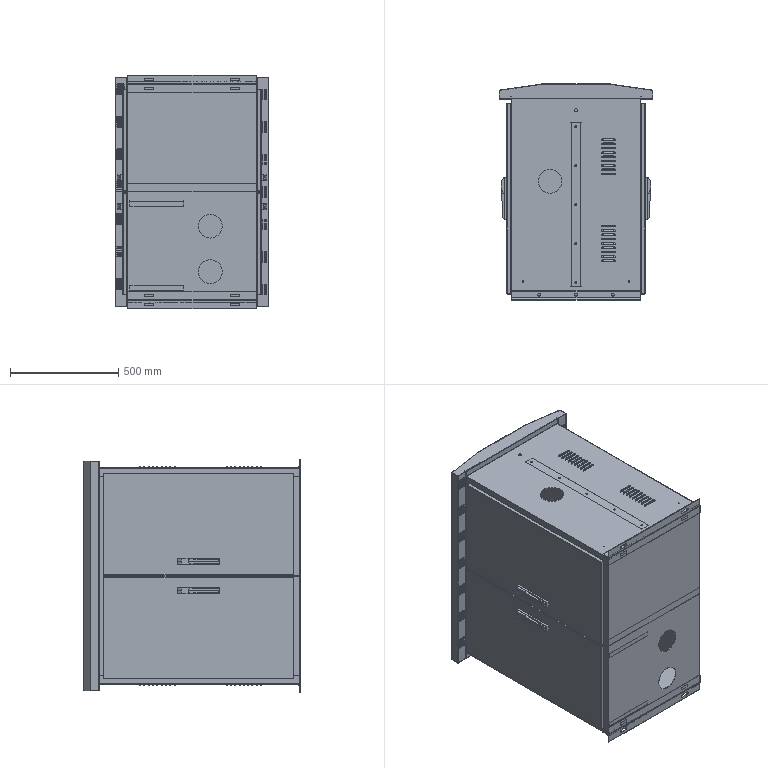Assembly | SolidWorks | mm | 61 component files | 65 solids | 4519 faces | box 710 x 1000 x 1080 mm | volume 12516403 mm3 | plane 2101 | cylinder 1978 | torus 176 | sphere 144 | spline 72 | cone 48 | commonest cylinder face diameters 4.5 x344 5.5 x332 4 x288 6 x222 4.473 x98 1.473 x98 9 x86 12 x56
Bill of materials:
CompensationChamberDoorPanel | 1 |  | Thin rectangular sheet panel with short perimeter return flanges; one large rectangular cutout near the top and a pattern of round holes below it.
CompositeSwitchMountingBeam100 | 2 |  | Long, narrow formed sheet bracket with a U/channel-type cross-section and flat extended end tabs, each tab carrying two elongated slots.
FrameLongitudinalBeamFive100 | 1 |  | Long open U-channel (open side up) formed from sheet, with pairs of small holes along both side walls.
FrameLongitudinalBeamFour01100 | 1 |  | Long open U-channel formed from sheet, with paired small holes along the side walls and holes near each end of the web.
FrameLongitudinalBeamOne01100 | 1 |  | Long L-section angle formed from sheet; one leg has five evenly spaced elongated slots, and that leg is slightly shorter than the other with trimmed corners at its ends.
FrameLongitudinalBeamSix100 | 1 |  | Long inverted U-channel (open side down) formed from sheet, with two holes at each end of the web and paired small holes along the side walls.
FrameLongitudinalBeamThree40001100 | 1 |  | Long plain L-section angle with a rounded bend; one leg carries five evenly spaced elongated slots.
FrameLongitudinalBeamTwo40001100 | 1 |  | Long inverted U-channel formed from sheet, with a row of evenly spaced round holes along the web and paired small holes along the side walls.
FrameTransverseBeamOne40001100 | 2 |  | Short, deep U-channel formed from sheet with rounded bends and rounded wall corners; two round holes near each end of one side wall.
FrameTransverseBeamTwo40001100 | 2 |  | Long, narrow formed sheet bracket with a hat/inverted-U profile and flat extended end tabs, each tab having two elongated slots; multiple round holes along the web.
FrontLeftDoorPanel100 | 1 |  | Thin flat rectangular plate with one rectangular slot near the centre of one long edge, flanked by two small round holes.
MS830-Lock | 4 | Plain Carbon Steel | Elongated solid, lever- or block-like body with a longitudinal groove along its length, a cylindrical boss partway along, a tapered section, and an angled/chamfered end.
FrontRightDoorPanel100 | 1 |  | Flat rectangular plate with a single rectangular slot near one long edge, centered along it, with one small round hole on each side of the slot.
FrontSealingPlate100 | 1 |  | Long, narrow, thin sheet panel. Both short ends have a slight downward bend or short lip. It has four larger round holes in a row near one end and four small corner holes, two at each end.
FuseGroupMountingBeam100 | 1 |  | Long U-channel bracket with rounded bend corners. The web extends past the flanges at both ends as flat tabs, and each tab has two elongated slots. Pairs of small round holes are spaced along the web.
GroundWireFixingBeam100 | 1 |  | Long U-channel bracket with rounded bends and extended end tabs, each tab with two elongated slots. Three larger round holes run along the web centerline, and one flange has a row of five small holes.
GB_INTERCHANGEABLE_PARTS_TM_EAI 4X4X594 | 4 |  | Straight, long angle-section (L-profile) bar with two legs that look equal. One leg has three round through-holes spaced along its length. The other leg has two slots, elongated along the length, one near each end.
InsulatorSYZ9-10Q100 | 4 |  | Solid body of revolution, roughly barrel-shaped. A raised cylindrical band in the middle sits between two tapered (frustum) ends, and each end face has a small central hole. The edges are slightly rounded.
LeftSidePlate400AType40001100 | 1 |  | Shallow rectangular sheet tray. Upturned side walls run along two opposite edges and end in small outward lips. The base has two groups of parallel louvers and one small round hole.
LowerCrossbar400AType40001100 | 1 |  | Sheet panel with a hat-shaped section: a flat web, two side walls bent at right angles, and short outward flanges. Both side walls have a rectangular notch at the same position partway along their length. Two large round holes sit near one side of the web.
MeteringChamberDoorPanel | 1 |  | Rectangular plate with four rectangular cutouts: one in the upper left and three stacked in a column on the right. It also has a small round hole near the top center and a pattern of one central hole with four small holes arranged in a cross around it.
MeteringChamberPartition400AType40001100 | 1 |  | Very thin flat rectangular plate with rounded corners. Three large round holes run in a column near one short edge. Small elongated slots run along both long edges, and four small round holes form a rectangular pattern.
MiddleCrossbar400AType40001100 | 2 |  | Long straight profile with a constant lipped C-channel section: a flat web, two flanges, and inward-angled lips with rounded ends. No holes are visible.
MoldedCaseMountingBeamOne100 | 4 |  | Long U-channel bracket with extended end tabs, each tab with two elongated slots. One flange has five small holes and the web has two small holes. A cylindrical boss with a chamfered end projects from the web into the inside of the channel.
MoldedCaseMountingBeamThree100 | 2 |  | Long U-channel bracket with rounded bends and extended end tabs, each tab with two elongated slots. The web has three pairs of small round holes along its centerline.
MoldedCaseMountingBeamTwo100 | 2 |  | Long, narrow formed channel (C-section) with rounded bends. The web is extended at both ends into tabs, and each tab has two slotted holes. Small round holes run along the web and the flange.
OutputN01400AType40001100 | 2 |  | Hat-profile formed bracket. Two outer mounting flanges are joined by short legs to an offset central web. Each flange has one round hole and the web has three.
RearCoverPlate100 | 1 |  | Thin, long rectangular plate with very shallow edge lips along the long sides. It has four small holes near the corners and a row of four larger round holes near one end.
RearLeftDoorPanel100 | 1 |  | Rectangular panel with a shallow folded perimeter edge (tray-like). It has a rectangular slot near one long edge, with a small round hole on each side of the slot.
RearRightDoorPanel100 | 1 |  | Rectangular panel with a shallow folded perimeter edge. It has a rectangular slot near the opposite long edge from unnamed part, with a small hole on each side.
RightSidePlate400AType40001100 | 1 |  | Shallow rectangular box-shaped cover with folded side walls. The top face has one large circular hole, one small hole, and two groups of parallel louvers or slots. Short flanges stick out past the walls along the long sides.
SmallDoorFrameOne100 | 4 |  | Long formed strip with a constant cross-section. The profile steps through several rounded bends: a hemmed J-hook at one end, two offset steps, and an upturned flange at the other end.
SmallDoorFrameTwo100 | 2 |  | Formed strip with the same kind of stepped multi-bend profile as unnamed part (hooked hem, two offsets, end flange), shown as a shorter piece.
TopCover01100 | 1 |  | Large formed panel with a faceted, arched cross-section (a central flat and two angled facets). Both side edges turn into narrow return flanges with small lips, and these returns carry repeated groups of small parallel slots or louvers.
TopCoverPlug01100 | 2 |  | Long formed strip with a flat top whose outline tapers at both ends (faceted, elongated hexagonal outline). A downturned leg runs along one edge and ends in a short stepped return.
UpperCrossbarFront400AType40001100 | 1 |  | Long L-angle with a rounded bend. One flange has a small rectangular notch at about mid-length.
UpperCrossbarRear400AType40001100 | 1 |  | Long L-angle with a rounded bend, oriented opposite to unnamed part. One flange has a small rectangular notch at about mid-length.
Mates:
1. coincident | LeftSidePlate400AType40001100-3 face at (890.554, 1085, -1.5) dir (0, 1, 0) | RightSidePlate400AType40001100-2 face at (293.554, 1085, 998.5) dir (0, 1, 0)
2. coincident | LeftSidePlate400AType40001100-3 face at (892.054, 1085, 0) dir (1, 0, 0) | RightSidePlate400AType40001100-2 face at (892.054, 1085, 958.5) dir (1, 0, 0)
3. coincident | LeftSidePlate400AType40001100-3 face at (292.054, 1085, 38.5) dir (-1, 0, 0) | UpperCrossbarRear400AType40001100-1 face at (292.054, 1087, 958.5) dir (-1, 0, 0)
4. width | LeftSidePlate400AType40001100-3 face at (890.554, 147, -1.5) dir (0, 0, -1) | RightSidePlate400AType40001100-2 face at (293.554, 147, 998.5) dir (0, 0, 1) | UpperCrossbarRear400AType40001100-1 face at (293.554, 1037, 958.5) dir (0, 0, 1) | UpperCrossbarRear400AType40001100-1 face at (293.554, 1037, 38.5) dir (0, 0, -1)
5. coincident | LeftSidePlate400AType40001100-3 face at (892.054, 1085, 0) dir (1, 0, 0) | UpperCrossbarFront400AType40001100-2 face at (892.054, 1087, 38.5) dir (1, 0, 0)
6. width | RightSidePlate400AType40001100-2 face at (293.554, 147, 998.5) dir (0, 0, 1) | LeftSidePlate400AType40001100-3 face at (890.554, 147, -1.5) dir (0, 0, -1) | UpperCrossbarFront400AType40001100-2 face at (890.554, 1037, 958.5) dir (0, 0, 1) | UpperCrossbarFront400AType40001100-2 face at (890.554, 1037, 38.5) dir (0, 0, -1)
7. coincident | LowerCrossbar400AType40001100-1 face at (292.054, 147, 38.5) dir (0, -1, 0) | RightSidePlate400AType40001100-2 face at (889.818, 147, 958.5) dir (0, -1, 0)
8. width | LeftSidePlate400AType40001100-3 face at (890.554, 147, -1.5) dir (0, 0, -1) | RightSidePlate400AType40001100-2 face at (293.554, 147, 998.5) dir (0, 0, 1) | LowerCrossbar400AType40001100-1 face at (892.054, 148.5, 958.5) dir (0, 0, 1) | LowerCrossbar400AType40001100-1 face at (892.054, 148.5, 38.5) dir (0, 0, -1)
9. width | RightSidePlate400AType40001100-2 face at (892.054, 1085, 958.5) dir (1, 0, 0) | RightSidePlate400AType40001100-2 face at (292.054, 1085, 997) dir (-1, 0, 0) | LowerCrossbar400AType40001100-1 face at (892.054, 148.5, 38.5) dir (1, 0, 0) | LowerCrossbar400AType40001100-1 face at (292.054, 148.5, 958.5) dir (-1, 0, 0)
10. width | TopCover01100-2/TopCoverPlug01100-1 face at (292.054, 1078.5, 1028.5) dir (0, 0, 1) | TopCover01100-2/TopCoverPlug01100-2 face at (892.054, 1078.5, -31.5) dir (0, 0, -1) | RightSidePlate400AType40001100-2 face at (293.554, 147, 998.5) dir (0, 0, 1) | LeftSidePlate400AType40001100-3 face at (890.554, 147, -1.5) dir (0, 0, -1)
11. width | TopCover01100-2/TopCover01100-1 face at (947.054, 1117, -31.5) dir (1, 0, 0) | TopCover01100-2/TopCover01100-1 face at (237.054, 1117, -31.5) dir (-1, 0, 0) | UpperCrossbarFront400AType40001100-2 face at (892.054, 1087, 38.5) dir (1, 0, 0) | UpperCrossbarRear400AType40001100-1 face at (292.054, 1087, 958.5) dir (-1, 0, 0)
12. coincident | assembly face at (474.554, -504, 592.5) dir (0, -1, 0) | assembly face at (464.554, -504, 400.5) dir (0, -1, 0)
13. coincident | UpperCrossbarFront400AType40001100-2 face at (892.054, 1087, 38.5) dir (1, 0, 0) | MiddleCrossbar400AType40001100-3 face at (892.054, 1038.5, 468.5) dir (1, 0, 0)
14. coincident | UpperCrossbarRear400AType40001100-1 face at (292.054, 1087, 958.5) dir (-1, 0, 0) | MiddleCrossbar400AType40001100-4 face at (292.054, 1038.5, 528.5) dir (-1, 0, 0)
15. coincident | LowerCrossbar400AType40001100-1 face at (277.554, 199, 958.5) dir (0, -1, 0) | MiddleCrossbar400AType40001100-4 face at (293.554, 199, 468.5) dir (0, -1, 0)
16. distance | TopCover01100-2/TopCover01100-1 face at (237.054, 1077, -31.5) dir (0, -1, 0) | LowerCrossbar400AType40001100-1 face at (292.054, 147, 38.5) dir (0, -1, 0)
17. distance | UpperCrossbarFront400AType40001100-2 face at (890.554, 1087, 38.5) dir (0, 1, 0) | TopCover01100-2/TopCover01100-1 face at (947.054, 1077, -31.5) dir (0, -1, 0)
18. coincident | UpperCrossbarRear400AType40001100-1 face at (277.554, 1037, 38.5) dir (0, -1, 0) | UpperCrossbarFront400AType40001100-2 face at (906.554, 1037, 958.5) dir (0, -1, 0)
19. coincident | LowerCrossbar400AType40001100-1 face at (892.054, 199, 958.5) dir (0, -1, 0) | MiddleCrossbar400AType40001100-3 face at (890.554, 199, 528.5) dir (0, -1, 0)
20. coincident | MiddleCrossbar400AType40001100-3 face at (902.554, 1038.5, 528.5) dir (0, 0, 1) | MiddleCrossbar400AType40001100-4 face at (281.554, 199, 528.5) dir (0, 0, 1)
21. parallel | TopCover01100-2/TopCover01100-1 face at (947.054, 1117, -31.5) dir (1, 0, 0) | MoldedCaseMountingBeamOne100-18 face at (618.554, 920.5, 992.375) dir (1, 0, 0)
22. coincident | MeteringChamberPartition400AType40001100-2 face at (567.054, 160.75, 505.125) dir (1, 0, 0) | FrameLongitudinalBeamFour01100-1 face at (567.054, 1082, 529.25) dir (-1, 0, 0)
23. width | MoldedCaseMountingBeamThree100-2 face at (618.554, 676, 494.125) dir (0, 0, 1) | MoldedCaseMountingBeamThree100-2 face at (618.554, 676, 3.625) dir (0, 0, -1) | FrameLongitudinalBeamSix100-2 face at (567.054, 154, 497.75) dir (0, 0, 1) | LeftSidePlate400AType40001100-3 face at (890.554, 147, 0) dir (0, 0, 1)
24. distance | GroundWireFixingBeam100-20 face at (618.554, 249.236, 992.375) dir (1, 0, 0) | OutputN01400AType40001100-2 face at (711.554, 244.236, 689.25) dir (-1, 0, 0)
25. coincident | assembly face at (438.554, -282.5, 1028.5) dir (0, 0, 1) | OutputN01400AType40001100-2 face at (670.554, 244.236, 725.25) dir (0, 0, 1)
26. width | MiddleCrossbar400AType40001100-4 face at (292.054, 1038.5, 528.5) dir (-1, 0, 0) | MiddleCrossbar400AType40001100-3 face at (892.054, 1038.5, 468.5) dir (1, 0, 0) | FrameLongitudinalBeamOne01100-2 face at (905.554, 1088.5, 537.25) dir (1, 0, 0) | FrameLongitudinalBeamOne01100-2 face at (278.554, 1088.5, 537.25) dir (-1, 0, 0)
27. coincident | TopCover01100-2/TopCover01100-1 face at (292.051, 1087, 1026.5) dir (0, 1, 0) | FrameLongitudinalBeamOne01100-2 face at (278.554, 1087, 501.75) dir (0, -1, 0)
28. width | FrameLongitudinalBeamOne01100-2 face at (297.554, 1048.5, 499.25) dir (0, 0, 1) | FrameLongitudinalBeamOne01100-2 face at (297.554, 1048.5, 497.75) dir (0, 0, -1) | LeftSidePlate400AType40001100-3 face at (890.554, 147, -1.5) dir (0, 0, -1) | RightSidePlate400AType40001100-2 face at (293.554, 147, 998.5) dir (0, 0, 1)
29. coincident | RightSidePlate400AType40001100-2 face at (293.554, 147, 997) dir (0, 0, -1) | FrameLongitudinalBeamTwo40001100-1 face at (617.054, 967, 997) dir (0, 0, 1)
30. distance | FrameLongitudinalBeamTwo40001100-1 face at (567.054, 207, 997) dir (0, -1, 0) | LowerCrossbar400AType40001100-1 face at (292.054, 147, 38.5) dir (0, -1, 0)
31. coincident | LowerCrossbar400AType40001100-1 face at (292.054, 148.5, 38.5) dir (0, 1, 0) | FrameLongitudinalBeamThree40001100-3 face at (889.554, 148.5, 497.75) dir (0, -1, 0)
32. coincident | FrameLongitudinalBeamOne01100-2 face at (297.554, 1048.5, 497.75) dir (0, 0, -1) | FrameLongitudinalBeamThree40001100-3 face at (889.554, 188.5, 497.75) dir (0, 0, -1)
33. width | FrameLongitudinalBeamThree40001100-3 face at (889.554, 148.5, 537.75) dir (1, 0, 0) | FrameLongitudinalBeamThree40001100-3 face at (294.554, 148.5, 537.75) dir (-1, 0, 0) | LowerCrossbar400AType40001100-1 face at (292.054, 148.5, 958.5) dir (-1, 0, 0) | LowerCrossbar400AType40001100-1 face at (892.054, 148.5, 38.5) dir (1, 0, 0)
34. coincident | FrameLongitudinalBeamThree40001100-3 face at (889.554, 188.5, 499.25) dir (0, 0, 1) | FrameLongitudinalBeamFour01100-1 face at (617.054, 155, 499.25) dir (0, 0, -1)
35. coincident | FrameLongitudinalBeamTwo40001100-1 face at (617.054, 967, 967) dir (1, 0, 0) | FrameLongitudinalBeamFour01100-1 face at (617.054, 155, 529.25) dir (1, 0, 0)
36. distance | FrameLongitudinalBeamFour01100-1 face at (567.054, 155, 499.25) dir (0, -1, 0) | FrameLongitudinalBeamThree40001100-3 face at (889.554, 150, 497.75) dir (0, 1, 0)
37. width | MoldedCaseMountingBeamOne100-18 face at (618.554, 880.5, 992.375) dir (0, 0, 1) | MoldedCaseMountingBeamOne100-18 face at (618.554, 880.5, 503.875) dir (0, 0, -1) | FrameLongitudinalBeamFour01100-1 face at (617.054, 155, 499.25) dir (0, 0, -1) | RightSidePlate400AType40001100-2 face at (293.554, 147, 997) dir (0, 0, -1)
38. coincident | MoldedCaseMountingBeamOne100-18 face at (617.054, 920.5, 992.375) dir (-1, 0, 0) | FrameLongitudinalBeamTwo40001100-1 face at (617.054, 967, 967) dir (1, 0, 0)
39. width | MeteringChamberPartition400AType40001100-2 face at (567.054, 1076.75, 505.125) dir (0, 0, -1) | MeteringChamberPartition400AType40001100-2 face at (567.054, 1076.75, 991.125) dir (0, 0, 1) | FrameLongitudinalBeamFour01100-1 face at (617.054, 155, 499.25) dir (0, 0, -1) | RightSidePlate400AType40001100-2 face at (293.554, 147, 997) dir (0, 0, -1)
40. width | LowerCrossbar400AType40001100-1 face at (277.554, 200.5, 958.5) dir (0, 1, 0) | UpperCrossbarRear400AType40001100-1 face at (277.554, 1037, 38.5) dir (0, -1, 0) | MeteringChamberPartition400AType40001100-2 face at (567.054, 160.75, 505.125) dir (0, -1, 0) | MeteringChamberPartition400AType40001100-2 face at (567.054, 1076.75, 505.125) dir (0, 1, 0)
41. coincident | FrameLongitudinalBeamTwo40001100-1 face at (617.054, 207, 967) dir (0, -1, 0) | FrameLongitudinalBeamFive100-2 face at (567.054, 207, 30) dir (0, -1, 0)
42. coincident | LeftSidePlate400AType40001100-3 face at (890.554, 147, 0) dir (0, 0, 1) | FrameLongitudinalBeamFive100-2 face at (567.054, 987, 0) dir (0, 0, -1)
43. coincident | FrameLongitudinalBeamTwo40001100-1 face at (617.054, 967, 967) dir (1, 0, 0) | FrameLongitudinalBeamFive100-2 face at (617.054, 207, 30) dir (1, 0, 0)
44. coincident | FrameLongitudinalBeamThree40001100-3 face at (889.554, 188.5, 497.75) dir (0, 0, -1) | FrameLongitudinalBeamSix100-2 face at (567.054, 154, 497.75) dir (0, 0, 1)
45. distance | FrameLongitudinalBeamSix100-2 face at (617.054, 154, 497.75) dir (0, -1, 0) | FrameLongitudinalBeamThree40001100-3 face at (889.554, 150, 497.75) dir (0, 1, 0)
46. coincident | MoldedCaseMountingBeamThree100-2 face at (617.054, 716, 494.125) dir (-1, 0, 0) | FrameLongitudinalBeamSix100-2 face at (617.054, 1081, 467.75) dir (1, 0, 0)
47. coincident | FrameLongitudinalBeamFive100-2 face at (617.054, 207, 30) dir (1, 0, 0) | FrameLongitudinalBeamSix100-2 face at (617.054, 1081, 467.75) dir (1, 0, 0)
48. coincident | FrameLongitudinalBeamFive100-2 face at (567.054, 987, 30) dir (-1, 0, 0) | CompositeSwitchMountingBeam100-7 face at (567.054, 674.236, 3.625) dir (1, 0, 0)
49. coincident | FrameLongitudinalBeamFive100-2 face at (567.054, 987, 30) dir (-1, 0, 0) | FuseGroupMountingBeam100-9 face at (567.054, 788.709, 3.625) dir (1, 0, 0)
50. coincident | CompositeSwitchMountingBeam100-7 face at (580.554, 676.473, 464.125) dir (0, 0, 1) | FuseGroupMountingBeam100-9 face at (580.554, 790.946, 464.125) dir (0, 0, 1)
51. distance | CompositeSwitchMountingBeam100-7 face at (580.554, 676.473, 33.625) dir (0, 1, 0) | FuseGroupMountingBeam100-9 face at (580.554, 746.473, 464.125) dir (0, -1, 0)
52. width | FrameLongitudinalBeamTwo40001100-1 face at (617.054, 967, 967) dir (1, 0, 0) | FrameLongitudinalBeamTwo40001100-1 face at (567.054, 207, 967) dir (-1, 0, 0) | RightSidePlate400AType40001100-2 face at (292.054, 1085, 997) dir (-1, 0, 0) | RightSidePlate400AType40001100-2 face at (892.054, 1085, 958.5) dir (1, 0, 0)
53. distance | FrameLongitudinalBeamFour01100-1 face at (567.054, 1082, 529.25) dir (0, 0, 1) | OutputN01400AType40001100-2 face at (670.554, 244.236, 579.25) dir (0, 0, -1)
54. parallel | LeftSidePlate400AType40001100-3 face at (890.554, 147, 0) dir (0, 0, 1) | FrameTransverseBeamOne40001100-2 face at (302.054, 193.5, 456.25) dir (0, 0, -1)
55. coincident | FrameTransverseBeamOne40001100-1 face at (302.054, 148.5, 65) dir (0, -1, 0) | FrameTransverseBeamOne40001100-2 face at (552.054, 148.5, 432.75) dir (0, -1, 0)
56. coincident | LowerCrossbar400AType40001100-1 face at (292.054, 148.5, 38.5) dir (0, 1, 0) | FrameTransverseBeamOne40001100-1 face at (302.054, 148.5, 65) dir (0, -1, 0)
57. distance | LeftSidePlate400AType40001100-3 face at (890.554, 147, 0) dir (0, 0, 1) | FrameTransverseBeamOne40001100-1 face at (552.054, 193.5, 40) dir (0, 0, -1)
58. distance | FrameLongitudinalBeamSix100-2 face at (567.054, 154, 497.75) dir (0, 0, 1) | FrameTransverseBeamOne40001100-2 face at (302.054, 193.5, 457.75) dir (0, 0, 1)
59. coincident | FrameTransverseBeamOne40001100-1 face at (302.054, 148.5, 40) dir (-1, 0, 0) | FrameTransverseBeamOne40001100-2 face at (302.054, 148.5, 457.75) dir (-1, 0, 0)
60. coincident | FrameTransverseBeamOne40001100-1 face at (552.054, 193.5, 65) dir (0, 1, 0) | FrameTransverseBeamTwo40001100-1 face at (349.554, 193.5, 43.375) dir (0, -1, 0)
61. width | FrameTransverseBeamOne40001100-1 face at (552.054, 193.5, 40) dir (0, 0, -1) | FrameTransverseBeamOne40001100-2 face at (302.054, 193.5, 457.75) dir (0, 0, 1) | FrameTransverseBeamTwo40001100-1 face at (317.554, 195, 454.375) dir (0, 0, 1) | FrameTransverseBeamTwo40001100-1 face at (317.554, 195, 43.375) dir (0, 0, -1)
62. coincident | FrameTransverseBeamOne40001100-2 face at (302.054, 193.5, 432.75) dir (0, 1, 0) | FrameTransverseBeamTwo40001100-2 face at (536.554, 193.5, 43.375) dir (0, -1, 0)
63. coincident | FrameTransverseBeamTwo40001100-1 face at (317.554, 195, 454.375) dir (0, 0, 1) | FrameTransverseBeamTwo40001100-2 face at (504.554, 195, 454.375) dir (0, 0, 1)
64. coincident | MiddleCrossbar400AType40001100-3 face at (890.554, 1038.5, 468.5) dir (-1, 0, 0) | SmallDoorFrameOne100-1 face at (890.554, 1037, 468.5) dir (1, 0, 0)
65. coincident | MiddleCrossbar400AType40001100-3 face at (902.554, 199, 468.5) dir (0, 0, -1) | SmallDoorFrameOne100-1 face at (857.554, 1037, 468.5) dir (0, 0, -1)
66. coincident | UpperCrossbarFront400AType40001100-2 face at (906.554, 1037, 958.5) dir (0, -1, 0) | SmallDoorFrameOne100-1 face at (856.054, 1037, 467.3) dir (0, 1, 0)
67. coincident | LeftSidePlate400AType40001100-3 face at (890.554, 1085, 0) dir (-1, 0, 0) | SmallDoorFrameOne100-2 face at (890.554, 741, 38.5) dir (1, 0, 0)
68. coincident | LeftSidePlate400AType40001100-3 face at (906.554, 1037, 38.5) dir (0, 0, 1) | SmallDoorFrameOne100-2 face at (857.554, 741, 38.5) dir (0, 0, 1)
69. coincident | SmallDoorFrameOne100-1 face at (889.054, 741, 471.2) dir (0, -1, 0) | SmallDoorFrameOne100-2 face at (856.054, 741, 39.7) dir (0, -1, 0)
70. coincident | UpperCrossbarFront400AType40001100-2 face at (890.554, 1087, 38.5) dir (-1, 0, 0) | SmallDoorFrameTwo100-3 face at (890.554, 1037, 38.5) dir (1, 0, 0)
71. coincident | UpperCrossbarFront400AType40001100-2 face at (906.554, 1037, 958.5) dir (0, -1, 0) | SmallDoorFrameTwo100-3 face at (857.554, 1037, 38.5) dir (0, -1, 0)
72. coincident | SmallDoorFrameOne100-2 face at (857.554, 741, 38.5) dir (0, 0, 1) | SmallDoorFrameTwo100-3 face at (856.054, 1035.8, 38.5) dir (0, 0, -1)
73. coincident | FrameLongitudinalBeamThree40001100-3 face at (889.554, 188.5, 497.75) dir (0, 0, -1) | FrontSealingPlate100-1 face at (622.304, 156.5, 497.75) dir (0, 0, 1)
74. width | LowerCrossbar400AType40001100-1 face at (292.054, 148.5, 38.5) dir (0, 1, 0) | FrameLongitudinalBeamOne01100-2 face at (278.554, 1088.5, 501.75) dir (0, 1, 0) | FrontSealingPlate100-1 face at (622.304, 1081.7, 490.75) dir (0, -1, 0) | FrontSealingPlate100-1 face at (885.304, 155.3, 490.75) dir (0, 1, 0)
75. width | FrameLongitudinalBeamSix100-2 face at (617.054, 1081, 467.75) dir (1, 0, 0) | MiddleCrossbar400AType40001100-3 face at (890.554, 1038.5, 468.5) dir (-1, 0, 0) | FrontSealingPlate100-1 face at (622.304, 1082.9, 496.55) dir (-1, 0, 0) | FrontSealingPlate100-1 face at (885.304, 1082.9, 490.75) dir (1, 0, 0)
76. coincident | FrameLongitudinalBeamThree40001100-3 face at (889.554, 188.5, 499.25) dir (0, 0, 1) | RearCoverPlate100-2 face at (562.554, 156.5, 499.25) dir (0, 0, -1)
77. width | MeteringChamberPartition400AType40001100-2 face at (565.554, 160.75, 505.125) dir (-1, 0, 0) | MiddleCrossbar400AType40001100-4 face at (293.554, 1038.5, 528.5) dir (1, 0, 0) | RearCoverPlate100-2 face at (562.554, 1082.9, 500.45) dir (1, 0, 0) | RearCoverPlate100-2 face at (296.554, 1082.9, 506.25) dir (-1, 0, 0)
78. width | RearCoverPlate100-2 face at (296.554, 155.3, 506.25) dir (0, 1, 0) | RearCoverPlate100-2 face at (562.554, 1081.7, 506.25) dir (0, -1, 0) | FrameLongitudinalBeamOne01100-2 face at (278.554, 1087, 501.75) dir (0, -1, 0) | FrameLongitudinalBeamThree40001100-3 face at (889.554, 150, 497.75) dir (0, 1, 0)
79. width | FrameTransverseBeamOne40001100-1 face at (302.054, 148.5, 40) dir (-1, 0, 0) | FrameTransverseBeamOne40001100-1 face at (552.054, 148.5, 40) dir (1, 0, 0) | FrameTransverseBeamTwo40001100-2 face at (540.554, 180, 67.375) dir (1, 0, 0) | FrameTransverseBeamTwo40001100-1 face at (313.554, 180, 430.375) dir (-1, 0, 0)
80. coincident | FrameLongitudinalBeamTwo40001100-1 face at (617.054, 967, 967) dir (1, 0, 0) | GroundWireFixingBeam100-20 face at (617.054, 249.236, 992.375) dir (-1, 0, 0)
81. coincident | FrameLongitudinalBeamTwo40001100-1 face at (617.054, 207, 967) dir (0, -1, 0) | GroundWireFixingBeam100-20 face at (603.554, 207, 532.875) dir (0, -1, 0)
82. width | OutputN01400AType40001100-2 face at (715.554, 214.236, 689.25) dir (0, -1, 0) | OutputN01400AType40001100-2 face at (715.554, 244.236, 689.25) dir (0, 1, 0) | GroundWireFixingBeam100-20 face at (603.554, 207, 532.875) dir (0, -1, 0) | GroundWireFixingBeam100-20 face at (603.554, 251.473, 963.375) dir (0, 1, 0)
83. coincident | InsulatorSYZ9-10Q100-1 face at (618.554, 229.236, 710.25) dir (-1, 0, 0) | InsulatorSYZ9-10Q100-2 face at (618.554, 229.236, 930.25) dir (-1, 0, 0)
84. coincident | InsulatorSYZ9-10Q100-2 face at (618.554, 229.236, 930.25) dir (-1, 0, 0) | InsulatorSYZ9-10Q100-3 face at (618.554, 229.236, 778.25) dir (-1, 0, 0)
85. coincident | InsulatorSYZ9-10Q100-2 face at (618.554, 229.236, 930.25) dir (-1, 0, 0) | InsulatorSYZ9-10Q100-4 face at (618.554, 229.236, 558.25) dir (-1, 0, 0)
86. coincident | GroundWireFixingBeam100-20 face at (618.554, 249.236, 992.375) dir (1, 0, 0) | InsulatorSYZ9-10Q100-2 face at (618.554, 229.236, 930.25) dir (-1, 0, 0)
87. concentric | InsulatorSYZ9-10Q100-3 face at (670.554, 229.236, 778.25) dir (1, 0, 0) r 2.6 | OutputN01400AType40001100-3 face at (664.554, 229.236, 778.25) dir (1, 0, 0) r 4.5
88. width | FrameLongitudinalBeamTwo40001100-1 face at (617.054, 967, 997) dir (0, 0, 1) | FrameLongitudinalBeamFour01100-1 face at (617.054, 155, 499.25) dir (0, 0, -1) | GroundWireFixingBeam100-20 face at (618.554, 209.236, 992.375) dir (0, 0, 1) | GroundWireFixingBeam100-20 face at (618.554, 209.236, 503.875) dir (0, 0, -1)
89. distance | RightSidePlate400AType40001100-2 face at (293.554, 147, 998.5) dir (0, 0, 1) | LeftSidePlate400AType40001100-3 face at (890.554, 147, -1.5) dir (0, 0, -1)
90. distance | LeftSidePlate400AType40001100-3 face at (906.554, 1037, 38.5) dir (0, 0, 1) | MiddleCrossbar400AType40001100-3 face at (902.554, 199, 468.5) dir (0, 0, -1)
91. coincident | MoldedCaseMountingBeamTwo100-3 face at (617.054, 436.5, 494.125) dir (-1, 0, 0) | FrameLongitudinalBeamFive100-2 face at (617.054, 207, 30) dir (1, 0, 0)
92. coincident | MoldedCaseMountingBeamThree100-2 face at (618.554, 676, 3.625) dir (0, 0, -1) | MoldedCaseMountingBeamTwo100-3 face at (618.554, 396.5, 3.625) dir (0, 0, -1)
93. coincident | MoldedCaseMountingBeamThree100-2 face at (618.554, 676, 3.625) dir (0, 0, -1) | CompositeSwitchMountingBeam100-7 face at (565.554, 634.236, 3.625) dir (0, 0, -1)
94. coincident | LeftSidePlate400AType40001100-3 face at (293.554, 1085, 38.5) dir (1, 0, 0) | SmallDoorFrameOne100-3 face at (293.554, 1037, 38.5) dir (-1, 0, 0)
95. coincident | LeftSidePlate400AType40001100-3 face at (277.554, 200.5, 38.5) dir (0, 0, 1) | SmallDoorFrameOne100-3 face at (326.554, 1037, 38.5) dir (0, 0, 1)
96. coincident | UpperCrossbarRear400AType40001100-1 face at (277.554, 1037, 38.5) dir (0, -1, 0) | SmallDoorFrameOne100-3 face at (328.054, 1037, 39.7) dir (0, 1, 0)
97. coincident | MiddleCrossbar400AType40001100-4 face at (293.554, 1038.5, 528.5) dir (1, 0, 0) | SmallDoorFrameOne100-4 face at (293.554, 741, 468.5) dir (-1, 0, 0)
98. coincident | MiddleCrossbar400AType40001100-4 face at (281.554, 1038.5, 468.5) dir (0, 0, -1) | SmallDoorFrameOne100-4 face at (326.554, 741, 468.5) dir (0, 0, -1)
99. coincident | SmallDoorFrameOne100-3 face at (328.054, 1037, 39.7) dir (0, 1, 0) | SmallDoorFrameOne100-4 face at (295.054, 1037, 471.2) dir (0, 1, 0)
100. coincident | UpperCrossbarRear400AType40001100-1 face at (293.554, 1087, 958.5) dir (1, 0, 0) | SmallDoorFrameTwo100-4 face at (293.554, 1037, 468.5) dir (-1, 0, 0)
101. coincident | UpperCrossbarRear400AType40001100-1 face at (277.554, 1037, 38.5) dir (0, -1, 0) | SmallDoorFrameTwo100-4 face at (326.554, 1037, 468.5) dir (0, -1, 0)
102. width | SmallDoorFrameTwo100-4 face at (328.054, 1035.8, 468.5) dir (0, 0, 1) | SmallDoorFrameTwo100-4 face at (295.054, 1039.7, 38.5) dir (0, 0, -1) | SmallDoorFrameOne100-4 face at (326.554, 741, 468.5) dir (0, 0, -1) | SmallDoorFrameOne100-3 face at (326.554, 1037, 38.5) dir (0, 0, 1)
103. distance | CompensationInnerDoorAssembly100-2/CompensationChamberDoorPanel-1 face at (346.554, 1015, 61) dir (0, 1, 0) | SmallDoorFrameTwo100-4 face at (345.354, 1017, 447.5) dir (0, -1, 0)
104. distance | SmallDoorFrameTwo100-4 face at (346.554, 1006.5, 70.5) dir (-1, 0, 0) | CompensationInnerDoorAssembly100-2/CompensationChamberDoorPanel-1 face at (326.554, 741, 446) dir (-1, 0, 0)
105. width | CompensationInnerDoorAssembly100-2/CompensationChamberDoorPanel-1 face at (346.554, 743.4, 61) dir (0, 0, -1) | CompensationInnerDoorAssembly100-2/CompensationChamberDoorPanel-1 face at (327.754, 743.4, 446) dir (0, 0, 1) | SmallDoorFrameOne100-3 face at (346.554, 1037, 58.5) dir (0, 0, 1) | SmallDoorFrameOne100-4 face at (346.554, 741, 448.5) dir (0, 0, -1)
106. distance | MeteringChamberDoorAssembly-1/MeteringChamberDoorPanel-1 face at (837.554, 1015, 446) dir (0, 1, 0) | SmallDoorFrameTwo100-3 face at (838.754, 1017, 59.5) dir (0, -1, 0)
107. width | SmallDoorFrameOne100-1 face at (837.554, 1037, 448.5) dir (0, 0, -1) | SmallDoorFrameOne100-2 face at (837.554, 741, 58.5) dir (0, 0, 1) | MeteringChamberDoorAssembly-1/MeteringChamberDoorPanel-1 face at (837.554, 743.4, 446) dir (0, 0, 1) | MeteringChamberDoorAssembly-1/MeteringChamberDoorPanel-1 face at (856.354, 743.4, 61) dir (0, 0, -1)
108. concentric | OutputN01400AType40001100-3 face at (664.554, 229.236, 930.25) dir (1, 0, 0) r 4.5 | InsulatorSYZ9-10Q100-2 face at (618.554, 229.236, 930.25) dir (-1, 0, 0) r 18
109. concentric | OutputN01400AType40001100-2 face at (664.554, 229.236, 710.25) dir (1, 0, 0) r 4.5 | InsulatorSYZ9-10Q100-1 face at (670.554, 229.236, 710.25) dir (1, 0, 0) r 2.6
110. concentric | OutputN01400AType40001100-2 face at (664.554, 229.236, 558.25) dir (1, 0, 0) r 4.5 | InsulatorSYZ9-10Q100-4 face at (670.554, 229.236, 558.25) dir (1, 0, 0) r 2.6
111. concentric | OutputN01400AType40001100-3 face at (664.554, 229.236, 778.25) dir (1, 0, 0) r 4.5 | InsulatorSYZ9-10Q100-3 face at (670.554, 229.236, 778.25) dir (1, 0, 0) r 2.6
112. distance | MeteringChamberDoorAssembly-1/MeteringChamberDoorPanel-1 face at (857.554, 741, 61) dir (1, 0, 0) | SmallDoorFrameTwo100-3 face at (837.554, 1006.5, 436.5) dir (1, 0, 0)
113. coincident | RightSidePlate400AType40001100-2 face at (293.554, 147, 997) dir (0, 0, -1) | hot-rolled equal angle gb-1 face at (295.054, 148.5, 997) dir (0, 0, 1)
114. width | RightSidePlate400AType40001100-2 face at (892.054, 1085, 958.5) dir (1, 0, 0) | RightSidePlate400AType40001100-2 face at (292.054, 1085, 997) dir (-1, 0, 0) | hot-rolled equal angle gb-1 face at (295.054, 151.166, 958.333) dir (-1, 0, 0) | hot-rolled equal angle gb-1 face at (889.054, 151.166, 958.333) dir (1, 0, 0)
115. coincident | RightSidePlate400AType40001100-2 face at (889.818, 148.5, 958.5) dir (0, 1, 0) | hot-rolled equal angle gb-1 face at (295.054, 148.5, 957) dir (0, -1, 0)
116. coincident | RightSidePlate400AType40001100-2 face at (293.554, 147, 998.5) dir (0, 0, 1) | hot-rolled equal angle gb-2 face at (889.054, 147, 998.5) dir (0, 0, -1)
117. coincident | hot-rolled equal angle gb-1 face at (889.054, 151.166, 958.333) dir (1, 0, 0) | hot-rolled equal angle gb-2 face at (889.054, 149.666, 1037.167) dir (1, 0, 0)
118. coincident | LowerCrossbar400AType40001100-1 face at (292.054, 147, 38.5) dir (0, -1, 0) | hot-rolled equal angle gb-2 face at (889.054, 147, 1038.5) dir (0, -1, 0)
119. coincident | LeftSidePlate400AType40001100-3 face at (890.554, 147, 0) dir (0, 0, 1) | hot-rolled equal angle gb-4 face at (889.054, 148.5, 0) dir (0, 0, -1)
120. coincident | LeftSidePlate400AType40001100-3 face at (890.554, 147, -1.5) dir (0, 0, -1) | hot-rolled equal angle gb-3 face at (295.054, 147, -1.5) dir (0, 0, 1)
121. coincident | LeftSidePlate400AType40001100-3 face at (294.291, 147, 38.5) dir (0, -1, 0) | hot-rolled equal angle gb-3 face at (295.054, 147, -41.5) dir (0, -1, 0)
122. coincident | LeftSidePlate400AType40001100-3 face at (294.291, 148.5, 38.5) dir (0, 1, 0) | hot-rolled equal angle gb-4 face at (889.054, 148.5, 40) dir (0, -1, 0)
123. coincident | hot-rolled equal angle gb-2 face at (889.054, 149.666, 1037.167) dir (1, 0, 0) | hot-rolled equal angle gb-3 face at (889.054, 149.666, -40.167) dir (1, 0, 0)
124. coincident | hot-rolled equal angle gb-1 face at (889.054, 151.166, 958.333) dir (1, 0, 0) | hot-rolled equal angle gb-4 face at (889.054, 151.166, 38.667) dir (1, 0, 0)
125. coincident | RightSidePlate400AType40001100-2 face at (892.054, 1085, 958.5) dir (1, 0, 0) | FrontLeftDoor-1/FrontLeftDoorPanel100-1 face at (892.054, 1055.5, 503.707) dir (-1, 0, 0)
126. distance | RightSidePlate400AType40001100-2 face at (293.554, 147, 998.5) dir (0, 0, 1) | FrontLeftDoor-1/FrontLeftDoorPanel100-1 face at (892.054, 176, 973.5) dir (0, 0, 1)
127. distance | TopCover01100-2/TopCover01100-1 face at (947.054, 1077, -31.5) dir (0, -1, 0) | FrontLeftDoor-1/FrontLeftDoorPanel100-1 face at (892.054, 1057, 973.5) dir (0, 1, 0)
128. coincident | UpperCrossbarFront400AType40001100-2 face at (892.054, 1087, 38.5) dir (1, 0, 0) | FrontRightDoor-1/FrontRightDoorPanel100-1 face at (892.054, 1055.5, 25.707) dir (-1, 0, 0)
129. distance | FrontRightDoor-1/FrontRightDoorPanel100-1 face at (892.054, 1057, 495.5) dir (0, 1, 0) | TopCover01100-2/TopCover01100-1 face at (947.054, 1077, -31.5) dir (0, -1, 0)
130. distance | LeftSidePlate400AType40001100-3 face at (890.554, 147, -1.5) dir (0, 0, -1) | FrontRightDoor-1/FrontRightDoorPanel100-1 face at (892.054, 1057, 23.5) dir (0, 0, -1)
131. coincident | UpperCrossbarRear400AType40001100-1 face at (292.054, 1087, 958.5) dir (-1, 0, 0) | RearLeftDoor-1/RearLeftDoorPanel100-1 face at (292.054, 1055.5, 493.293) dir (1, 0, 0)
132. distance | RearLeftDoor-1/RearLeftDoorPanel100-1 face at (292.054, 176, 23.5) dir (0, 0, -1) | LeftSidePlate400AType40001100-3 face at (890.554, 147, -1.5) dir (0, 0, -1)
133. distance | TopCover01100-2/TopCover01100-1 face at (237.054, 1077, -31.5) dir (0, -1, 0) | RearLeftDoor-1/RearLeftDoorPanel100-1 face at (292.054, 1057, 23.5) dir (0, 1, 0)
134. coincident | UpperCrossbarRear400AType40001100-1 face at (292.054, 1087, 958.5) dir (-1, 0, 0) | RearRightDoor-1/RearRightDoorPanel100-1 face at (292.054, 1055.5, 971.293) dir (1, 0, 0)
135. distance | TopCover01100-2/TopCover01100-1 face at (237.054, 1077, -31.5) dir (0, -1, 0) | RearRightDoor-1/RearRightDoorPanel100-1 face at (292.054, 1057, 501.5) dir (0, 1, 0)
136. distance | RearRightDoor-1/RearRightDoorPanel100-1 face at (292.054, 1057, 973.5) dir (0, 0, 1) | RightSidePlate400AType40001100-2 face at (293.554, 147, 998.5) dir (0, 0, 1)
137. coincident | FrontLeftDoorPanel100-1 face at (0, 881, -1.5) dir (0, 0, -1) | MS830-Lock-1 face at (-421, 342.25, -1.5) dir (0, 0, 1)
138. concentric | FrontLeftDoorPanel100-1 face at (-407, 525.75, 0) dir (0, 0, -1) r 3 | MS830-Lock-1 face at (-407, 525.75, -11.5) dir (0, 0, 1) r 3
139. coincident | FrontLeftDoorPanel100-1 edge at (-407, 355.25, -1.5) dir (0, 0, -1) r 3 | MS830-Lock-1 face at (-407, 355.25, -11.5) dir (0, 0, 1) r 3
140. coincident | FrontRightDoorPanel100-1 face at (0, 881, -1.5) dir (0, 0, -1) | MS830-Lock-1 face at (-79, 342.25, -1.5) dir (0, 0, 1)
141. concentric | FrontRightDoorPanel100-1 face at (-65, 525.75, 0) dir (0, 0, -1) r 3 | MS830-Lock-1 face at (-65, 525.75, -11.5) dir (0, 0, 1) r 3
142. concentric | FrontRightDoorPanel100-1 face at (-65, 355.25, 0) dir (0, 0, -1) r 3 | MS830-Lock-1 face at (-65, 355.25, -11.5) dir (0, 0, 1) r 3
143. coincident | RearLeftDoorPanel100-1 face at (0, 881, -1.5) dir (0, 0, -1) | MS830-Lock-1 face at (-421, 342.25, -1.5) dir (0, 0, 1)
144. concentric | RearLeftDoorPanel100-1 face at (-407, 525.75, 0) dir (0, 0, -1) r 3 | MS830-Lock-1 face at (-407, 525.75, -11.5) dir (0, 0, 1) r 3
145. coincident | RearLeftDoorPanel100-1 face at (-407, 355.25, 0) dir (0, 0, -1) r 3 | MS830-Lock-1 edge at (-407, 355.25, -1.5) dir (0, 0, 1) r 3
146. coincident | RearRightDoorPanel100-1 face at (0, 881, -1.5) dir (0, 0, -1) | MS830-Lock-1 face at (-79, 342.25, -1.5) dir (0, 0, 1)
147. concentric | RearRightDoorPanel100-1 face at (-65, 525.75, 0) dir (0, 0, -1) r 3 | MS830-Lock-1 face at (-65, 525.75, -11.5) dir (0, 0, 1) r 3
148. coincident | RearRightDoorPanel100-1 edge at (-65, 355.25, -1.5) dir (0, 0, -1) r 3 | MS830-Lock-1 face at (-65, 355.25, -11.5) dir (0, 0, 1) r 3
149. coincident | TopCoverPlug01100-1 face at (625.285, 42.2, -228.584) dir (0, 0, -1) | TopCover01100-1 face at (678.048, 42.937, -228.584) dir (0, 0, -1)
150. coincident | TopCoverPlug01100-2 face at (25.285, 42.2, 831.416) dir (0, 0, 1) | TopCover01100-1 face at (678.048, 42.937, 831.416) dir (0, 0, 1)
151. coincident | TopCover01100-1 face at (-29.715, 40.7, 831.416) dir (0, -1, 0) | TopCoverPlug01100-1 face at (625.285, 40.7, -200.824) dir (0, -1, 0)
152. width | TopCoverPlug01100-1 face at (625.285, 42.2, -228.584) dir (1, 0, 0) | TopCoverPlug01100-1 face at (25.285, 42.2, -228.584) dir (-1, 0, 0) | TopCover01100-1 face at (-29.715, 80.7, 831.416) dir (-1, 0, 0) | TopCover01100-1 face at (680.285, 80.7, 831.416) dir (1, 0, 0)
153. width | TopCoverPlug01100-2 face at (25.285, 50.7, 801.42) dir (-1, 0, 0) | TopCoverPlug01100-2 face at (625.285, 50.7, 794.92) dir (1, 0, 0) | TopCover01100-1 face at (680.285, 80.7, 831.416) dir (1, 0, 0) | TopCover01100-1 face at (-29.715, 80.7, 831.416) dir (-1, 0, 0)
154. coincident | TopCover01100-1 face at (-29.715, 40.7, 831.416) dir (0, -1, 0) | TopCoverPlug01100-2 face at (25.285, 40.7, 803.656) dir (0, -1, 0)
155. coincident | TopCover01100-1 face at (678.048, 42.937, -228.584) dir (0, 0, -1) | TopCoverPlug01100-1 face at (625.285, 42.2, -228.584) dir (0, 0, -1)